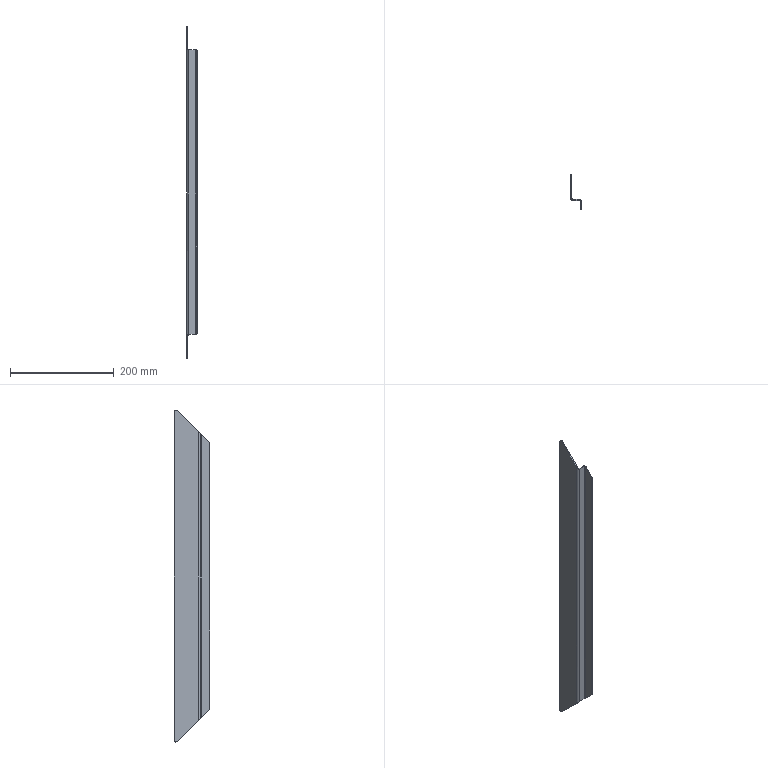Component | SolidWorks | BoxWelding-1_FrontAndRearPlate4-1 | 1 solid | 25 faces | box 20 x 68 x 641.51 mm | volume 96064 mm3 | plane 14 | cylinder 7 | spline 4 | commonest cylinder face diameters 6 x3 8 x2 4 x2
STEP:
#1=COLOUR_RGB('',0.7922,0.8196,0.9333);
#2=FILL_AREA_STYLE_COLOUR('',#1);
#3=FILL_AREA_STYLE('',(#2));
#4=SURFACE_STYLE_FILL_AREA(#3);
#5=SURFACE_SIDE_STYLE('',(#4));
#6=SURFACE_STYLE_USAGE(.BOTH.,#5);
#7=PRESENTATION_STYLE_ASSIGNMENT((#6));
#8=CARTESIAN_POINT('',(-8.991,51.201,-8.691));
#9=VERTEX_POINT('',#8);
#10=CARTESIAN_POINT('',(-8.991,51.117,-8.656));
#11=VERTEX_POINT('',#10);
#12=CARTESIAN_POINT('',(-8.991,51.201,-8.573));
#13=DIRECTION('',(-1.,-0.,-0.));
#14=DIRECTION('',(0.,0.,1.));
#15=AXIS2_PLACEMENT_3D('',#12,#13,#14);
#16=CIRCLE('',#15,0.1181);
#17=EDGE_CURVE('',#9,#11,#16,.T.);
#18=ORIENTED_EDGE('',*,*,#17,.F.);
#19=CARTESIAN_POINT('',(-8.913,51.201,-8.691));
#20=VERTEX_POINT('',#19);
#21=CARTESIAN_POINT('',(-8.991,51.201,-8.691));
#22=DIRECTION('',(1.,0.,0.));
#23=VECTOR('',#22,39.37);
#24=LINE('',#21,#23);
#25=EDGE_CURVE('',#9,#20,#24,.T.);
#26=ORIENTED_EDGE('',*,*,#25,.T.);
#27=CARTESIAN_POINT('',(-8.913,51.117,-8.656));
#28=VERTEX_POINT('',#27);
#29=CARTESIAN_POINT('',(-8.913,51.201,-8.573));
#30=DIRECTION('',(1.,0.,0.));
#31=DIRECTION('',(0.,0.,1.));
#32=AXIS2_PLACEMENT_3D('',#29,#30,#31);
#33=CIRCLE('',#32,0.1181);
#34=EDGE_CURVE('',#28,#20,#33,.T.);
#35=ORIENTED_EDGE('',*,*,#34,.F.);
#36=CARTESIAN_POINT('',(-8.913,51.117,-8.656));
#37=DIRECTION('',(1.,0.,0.));
#38=VECTOR('',#37,39.37);
#39=LINE('',#36,#38);
#40=EDGE_CURVE('',#11,#28,#39,.T.);
#41=ORIENTED_EDGE('',*,*,#40,.F.);
#42=EDGE_LOOP('',(#18,#26,#35,#41));
#43=FACE_OUTER_BOUND('',#42,.T.);
#44=CARTESIAN_POINT('',(-8.991,51.201,-8.573));
#45=DIRECTION('',(1.,0.,0.));
#46=DIRECTION('',(0.,-0.,-1.));
#47=AXIS2_PLACEMENT_3D('',#44,#45,#46);
#48=CYLINDRICAL_SURFACE('',#47,0.1181);
#49=ADVANCED_FACE('',(#43),#48,.T.);
#50=CARTESIAN_POINT('',(-8.834,49.35,14.764));
#51=VERTEX_POINT('',#50);
#52=CARTESIAN_POINT('',(-8.834,49.35,-6.889));
#53=VERTEX_POINT('',#52);
#54=CARTESIAN_POINT('',(-8.834,49.35,-8.858));
#55=DIRECTION('',(0.,-0.,-1.));
#56=VECTOR('',#55,39.37);
#57=LINE('',#54,#56);
#58=EDGE_CURVE('',#51,#53,#57,.T.);
#59=ORIENTED_EDGE('',*,*,#58,.T.);
#60=CARTESIAN_POINT('',(-8.361,49.35,-6.889));
#61=VERTEX_POINT('',#60);
#62=CARTESIAN_POINT('',(-8.913,49.35,-6.889));
#63=DIRECTION('',(-1.,-0.,-0.));
#64=VECTOR('',#63,39.37);
#65=LINE('',#62,#64);
#66=EDGE_CURVE('',#61,#53,#65,.T.);
#67=ORIENTED_EDGE('',*,*,#66,.F.);
#68=CARTESIAN_POINT('',(-8.361,49.35,14.764));
#69=VERTEX_POINT('',#68);
#70=CARTESIAN_POINT('',(-8.361,49.35,16.733));
#71=DIRECTION('',(0.,-0.,-1.));
#72=VECTOR('',#71,39.37);
#73=LINE('',#70,#72);
#74=EDGE_CURVE('',#69,#61,#73,.T.);
#75=ORIENTED_EDGE('',*,*,#74,.F.);
#76=CARTESIAN_POINT('',(-8.913,49.35,14.764));
#77=DIRECTION('',(1.,0.,0.));
#78=VECTOR('',#77,39.37);
#79=LINE('',#76,#78);
#80=EDGE_CURVE('',#51,#69,#79,.T.);
#81=ORIENTED_EDGE('',*,*,#80,.F.);
#82=EDGE_LOOP('',(#59,#67,#75,#81));
#83=FACE_OUTER_BOUND('',#82,.T.);
#84=CARTESIAN_POINT('',(-8.913,49.35,-8.858));
#85=DIRECTION('',(0.,-1.,0.));
#86=DIRECTION('',(1.,0.,0.));
#87=AXIS2_PLACEMENT_3D('',#84,#85,#86);
#88=PLANE('',#87);
#89=ADVANCED_FACE('',(#83),#88,.T.);
#90=CARTESIAN_POINT('',(-8.361,49.429,-6.889));
#91=VERTEX_POINT('',#90);
#92=CARTESIAN_POINT('',(-8.834,49.429,-6.889));
#93=VERTEX_POINT('',#92);
#94=CARTESIAN_POINT('',(-8.913,49.429,-6.889));
#95=DIRECTION('',(-1.,-0.,-0.));
#96=VECTOR('',#95,39.37);
#97=LINE('',#94,#96);
#98=EDGE_CURVE('',#91,#93,#97,.T.);
#99=ORIENTED_EDGE('',*,*,#98,.T.);
#100=CARTESIAN_POINT('',(-8.834,49.429,14.764));
#101=VERTEX_POINT('',#100);
#102=CARTESIAN_POINT('',(-8.834,49.429,16.733));
#103=DIRECTION('',(0.,-0.,-1.));
#104=VECTOR('',#103,39.37);
#105=LINE('',#102,#104);
#106=EDGE_CURVE('',#101,#93,#105,.T.);
#107=ORIENTED_EDGE('',*,*,#106,.F.);
#108=CARTESIAN_POINT('',(-8.361,49.429,14.764));
#109=VERTEX_POINT('',#108);
#110=CARTESIAN_POINT('',(-8.913,49.429,14.764));
#111=DIRECTION('',(1.,0.,0.));
#112=VECTOR('',#111,39.37);
#113=LINE('',#110,#112);
#114=EDGE_CURVE('',#101,#109,#113,.T.);
#115=ORIENTED_EDGE('',*,*,#114,.T.);
#116=CARTESIAN_POINT('',(-8.361,49.429,16.733));
#117=DIRECTION('',(0.,-0.,-1.));
#118=VECTOR('',#117,39.37);
#119=LINE('',#116,#118);
#120=EDGE_CURVE('',#109,#91,#119,.T.);
#121=ORIENTED_EDGE('',*,*,#120,.T.);
#122=EDGE_LOOP('',(#99,#107,#115,#121));
#123=FACE_OUTER_BOUND('',#122,.T.);
#124=CARTESIAN_POINT('',(-8.913,49.429,-8.858));
#125=DIRECTION('',(0.,-1.,0.));
#126=DIRECTION('',(1.,0.,0.));
#127=AXIS2_PLACEMENT_3D('',#124,#125,#126);
#128=PLANE('',#127);
#129=ADVANCED_FACE('',(#123),#128,.F.);
#130=CARTESIAN_POINT('',(-8.991,51.319,16.448));
#131=VERTEX_POINT('',#130);
#132=CARTESIAN_POINT('',(-8.991,51.319,-8.573));
#133=VERTEX_POINT('',#132);
#134=CARTESIAN_POINT('',(-8.991,51.319,-8.858));
#135=DIRECTION('',(0.,-0.,-1.));
#136=VECTOR('',#135,39.37);
#137=LINE('',#134,#136);
#138=EDGE_CURVE('',#131,#133,#137,.T.);
#139=ORIENTED_EDGE('',*,*,#138,.T.);
#140=CARTESIAN_POINT('',(-8.991,51.201,-8.573));
#141=DIRECTION('',(-1.,-0.,-0.));
#142=DIRECTION('',(0.,0.,1.));
#143=AXIS2_PLACEMENT_3D('',#140,#141,#142);
#144=CIRCLE('',#143,0.1181);
#145=EDGE_CURVE('',#133,#9,#144,.T.);
#146=ORIENTED_EDGE('',*,*,#145,.T.);
#147=ORIENTED_EDGE('',*,*,#17,.T.);
#148=CARTESIAN_POINT('',(-8.991,49.508,-7.047));
#149=VERTEX_POINT('',#148);
#150=CARTESIAN_POINT('',(-8.991,37.539,4.922));
#151=DIRECTION('',(-0.,0.7071,-0.7071));
#152=VECTOR('',#151,39.37);
#153=LINE('',#150,#152);
#154=EDGE_CURVE('',#149,#11,#153,.T.);
#155=ORIENTED_EDGE('',*,*,#154,.F.);
#156=CARTESIAN_POINT('',(-8.991,49.508,14.922));
#157=VERTEX_POINT('',#156);
#158=CARTESIAN_POINT('',(-8.991,49.508,-8.858));
#159=DIRECTION('',(-0.,0.,1.));
#160=VECTOR('',#159,39.37);
#161=LINE('',#158,#160);
#162=EDGE_CURVE('',#149,#157,#161,.T.);
#163=ORIENTED_EDGE('',*,*,#162,.T.);
#164=CARTESIAN_POINT('',(-8.991,51.117,16.531));
#165=VERTEX_POINT('',#164);
#166=CARTESIAN_POINT('',(-8.991,50.335,15.749));
#167=DIRECTION('',(0.,-0.7071,-0.7071));
#168=VECTOR('',#167,39.37);
#169=LINE('',#166,#168);
#170=EDGE_CURVE('',#165,#157,#169,.T.);
#171=ORIENTED_EDGE('',*,*,#170,.F.);
#172=CARTESIAN_POINT('',(-8.991,51.201,16.448));
#173=DIRECTION('',(-1.,-0.,-0.));
#174=DIRECTION('',(0.,0.,1.));
#175=AXIS2_PLACEMENT_3D('',#172,#173,#174);
#176=CIRCLE('',#175,0.1181);
#177=EDGE_CURVE('',#165,#131,#176,.T.);
#178=ORIENTED_EDGE('',*,*,#177,.T.);
#179=EDGE_LOOP('',(#139,#146,#147,#155,#163,#171,#178));
#180=FACE_OUTER_BOUND('',#179,.T.);
#181=CARTESIAN_POINT('',(-8.991,49.35,16.733));
#182=DIRECTION('',(-1.,-0.,-0.));
#183=DIRECTION('',(-0.,0.,1.));
#184=AXIS2_PLACEMENT_3D('',#181,#182,#183);
#185=PLANE('',#184);
#186=ADVANCED_FACE('',(#180),#185,.T.);
#187=CARTESIAN_POINT('',(-8.913,49.508,-7.047));
#188=VERTEX_POINT('',#187);
#189=CARTESIAN_POINT('',(-8.913,37.539,4.922));
#190=DIRECTION('',(-0.,0.7071,-0.7071));
#191=VECTOR('',#190,39.37);
#192=LINE('',#189,#191);
#193=EDGE_CURVE('',#188,#28,#192,.T.);
#194=ORIENTED_EDGE('',*,*,#193,.T.);
#195=ORIENTED_EDGE('',*,*,#34,.T.);
#196=CARTESIAN_POINT('',(-8.913,51.319,-8.573));
#197=VERTEX_POINT('',#196);
#198=CARTESIAN_POINT('',(-8.913,51.201,-8.573));
#199=DIRECTION('',(1.,0.,0.));
#200=DIRECTION('',(0.,0.,1.));
#201=AXIS2_PLACEMENT_3D('',#198,#199,#200);
#202=CIRCLE('',#201,0.1181);
#203=EDGE_CURVE('',#20,#197,#202,.T.);
#204=ORIENTED_EDGE('',*,*,#203,.T.);
#205=CARTESIAN_POINT('',(-8.913,51.319,16.448));
#206=VERTEX_POINT('',#205);
#207=CARTESIAN_POINT('',(-8.913,51.319,16.733));
#208=DIRECTION('',(0.,-0.,-1.));
#209=VECTOR('',#208,39.37);
#210=LINE('',#207,#209);
#211=EDGE_CURVE('',#206,#197,#210,.T.);
#212=ORIENTED_EDGE('',*,*,#211,.F.);
#213=CARTESIAN_POINT('',(-8.913,51.117,16.531));
#214=VERTEX_POINT('',#213);
#215=CARTESIAN_POINT('',(-8.913,51.201,16.448));
#216=DIRECTION('',(1.,0.,0.));
#217=DIRECTION('',(0.,0.,1.));
#218=AXIS2_PLACEMENT_3D('',#215,#216,#217);
#219=CIRCLE('',#218,0.1181);
#220=EDGE_CURVE('',#206,#214,#219,.T.);
#221=ORIENTED_EDGE('',*,*,#220,.T.);
#222=CARTESIAN_POINT('',(-8.913,49.508,14.922));
#223=VERTEX_POINT('',#222);
#224=CARTESIAN_POINT('',(-8.913,50.335,15.749));
#225=DIRECTION('',(0.,-0.7071,-0.7071));
#226=VECTOR('',#225,39.37);
#227=LINE('',#224,#226);
#228=EDGE_CURVE('',#214,#223,#227,.T.);
#229=ORIENTED_EDGE('',*,*,#228,.T.);
#230=CARTESIAN_POINT('',(-8.913,49.508,-8.858));
#231=DIRECTION('',(-0.,0.,1.));
#232=VECTOR('',#231,39.37);
#233=LINE('',#230,#232);
#234=EDGE_CURVE('',#188,#223,#233,.T.);
#235=ORIENTED_EDGE('',*,*,#234,.F.);
#236=EDGE_LOOP('',(#194,#195,#204,#212,#221,#229,#235));
#237=FACE_OUTER_BOUND('',#236,.T.);
#238=CARTESIAN_POINT('',(-8.913,49.35,16.733));
#239=DIRECTION('',(-1.,-0.,-0.));
#240=DIRECTION('',(-0.,0.,1.));
#241=AXIS2_PLACEMENT_3D('',#238,#239,#240);
#242=PLANE('',#241);
#243=ADVANCED_FACE('',(#237),#242,.F.);
#244=ORIENTED_EDGE('',*,*,#162,.F.);
#245=CARTESIAN_POINT('',(-8.834,49.35,-6.889));
#246=CARTESIAN_POINT('',(-8.926,49.35,-6.889));
#247=CARTESIAN_POINT('',(-8.991,49.416,-6.954));
#248=CARTESIAN_POINT('',(-8.991,49.508,-7.047));
#249=(BOUNDED_CURVE()B_SPLINE_CURVE(3,(#245,#246,#247,#248),.UNSPECIFIED.,.F.,.T.)B_SPLINE_CURVE_WITH_KNOTS((4,4),(3.142,4.712),.UNSPECIFIED.)CURVE()GEOMETRIC_REPRESENTATION_ITEM()RATIONAL_B_SPLINE_CURVE((1.,0.8047,0.8047,1.))REPRESENTATION_ITEM(''));
#250=EDGE_CURVE('',#53,#149,#249,.T.);
#251=ORIENTED_EDGE('',*,*,#250,.F.);
#252=ORIENTED_EDGE('',*,*,#58,.F.);
#253=CARTESIAN_POINT('',(-8.991,49.508,14.922));
#254=CARTESIAN_POINT('',(-8.991,49.416,14.83));
#255=CARTESIAN_POINT('',(-8.926,49.35,14.764));
#256=CARTESIAN_POINT('',(-8.834,49.35,14.764));
#257=(BOUNDED_CURVE()B_SPLINE_CURVE(3,(#253,#254,#255,#256),.UNSPECIFIED.,.F.,.T.)B_SPLINE_CURVE_WITH_KNOTS((4,4),(4.712,6.283),.UNSPECIFIED.)CURVE()GEOMETRIC_REPRESENTATION_ITEM()RATIONAL_B_SPLINE_CURVE((1.,0.8047,0.8047,1.))REPRESENTATION_ITEM(''));
#258=EDGE_CURVE('',#157,#51,#257,.T.);
#259=ORIENTED_EDGE('',*,*,#258,.F.);
#260=EDGE_LOOP('',(#244,#251,#252,#259));
#261=FACE_OUTER_BOUND('',#260,.T.);
#262=CARTESIAN_POINT('',(-8.834,49.508,-8.858));
#263=DIRECTION('',(0.,-0.,-1.));
#264=DIRECTION('',(0.,-1.,0.));
#265=AXIS2_PLACEMENT_3D('',#262,#263,#264);
#266=CYLINDRICAL_SURFACE('',#265,0.1575);
#267=ADVANCED_FACE('',(#261),#266,.T.);
#268=CARTESIAN_POINT('',(-8.834,49.429,-6.889));
#269=CARTESIAN_POINT('',(-8.88,49.429,-6.889));
#270=CARTESIAN_POINT('',(-8.913,49.462,-6.954));
#271=CARTESIAN_POINT('',(-8.913,49.508,-7.047));
#272=(BOUNDED_CURVE()B_SPLINE_CURVE(3,(#268,#269,#270,#271),.UNSPECIFIED.,.F.,.T.)B_SPLINE_CURVE_WITH_KNOTS((4,4),(3.142,4.712),.UNSPECIFIED.)CURVE()GEOMETRIC_REPRESENTATION_ITEM()RATIONAL_B_SPLINE_CURVE((1.,0.8047,0.8047,1.))REPRESENTATION_ITEM(''));
#273=EDGE_CURVE('',#93,#188,#272,.T.);
#274=ORIENTED_EDGE('',*,*,#273,.T.);
#275=ORIENTED_EDGE('',*,*,#234,.T.);
#276=CARTESIAN_POINT('',(-8.913,49.508,14.922));
#277=CARTESIAN_POINT('',(-8.913,49.462,14.83));
#278=CARTESIAN_POINT('',(-8.88,49.429,14.764));
#279=CARTESIAN_POINT('',(-8.834,49.429,14.764));
#280=(BOUNDED_CURVE()B_SPLINE_CURVE(3,(#276,#277,#278,#279),.UNSPECIFIED.,.F.,.T.)B_SPLINE_CURVE_WITH_KNOTS((4,4),(4.712,6.283),.UNSPECIFIED.)CURVE()GEOMETRIC_REPRESENTATION_ITEM()RATIONAL_B_SPLINE_CURVE((1.,0.8047,0.8047,1.))REPRESENTATION_ITEM(''));
#281=EDGE_CURVE('',#223,#101,#280,.T.);
#282=ORIENTED_EDGE('',*,*,#281,.T.);
#283=ORIENTED_EDGE('',*,*,#106,.T.);
#284=EDGE_LOOP('',(#274,#275,#282,#283));
#285=FACE_OUTER_BOUND('',#284,.T.);
#286=CARTESIAN_POINT('',(-8.834,49.508,-8.858));
#287=DIRECTION('',(0.,-0.,-1.));
#288=DIRECTION('',(0.,-1.,0.));
#289=AXIS2_PLACEMENT_3D('',#286,#287,#288);
#290=CYLINDRICAL_SURFACE('',#289,0.07874);
#291=ADVANCED_FACE('',(#285),#290,.F.);
#292=CARTESIAN_POINT('',(-8.204,49.272,-6.811));
#293=VERTEX_POINT('',#292);
#294=CARTESIAN_POINT('',(-8.204,49.272,14.686));
#295=VERTEX_POINT('',#294);
#296=CARTESIAN_POINT('',(-8.204,49.272,16.733));
#297=DIRECTION('',(-0.,0.,1.));
#298=VECTOR('',#297,39.37);
#299=LINE('',#296,#298);
#300=EDGE_CURVE('',#293,#295,#299,.T.);
#301=ORIENTED_EDGE('',*,*,#300,.F.);
#302=CARTESIAN_POINT('',(-8.361,49.429,-6.889));
#303=CARTESIAN_POINT('',(-8.269,49.429,-6.889));
#304=CARTESIAN_POINT('',(-8.204,49.364,-6.857));
#305=CARTESIAN_POINT('',(-8.204,49.272,-6.811));
#306=(BOUNDED_CURVE()B_SPLINE_CURVE(3,(#302,#303,#304,#305),.UNSPECIFIED.,.F.,.T.)B_SPLINE_CURVE_WITH_KNOTS((4,4),(3.142,4.712),.UNSPECIFIED.)CURVE()GEOMETRIC_REPRESENTATION_ITEM()RATIONAL_B_SPLINE_CURVE((1.,0.8047,0.8047,1.))REPRESENTATION_ITEM(''));
#307=EDGE_CURVE('',#91,#293,#306,.T.);
#308=ORIENTED_EDGE('',*,*,#307,.F.);
#309=ORIENTED_EDGE('',*,*,#120,.F.);
#310=CARTESIAN_POINT('',(-8.204,49.272,14.686));
#311=CARTESIAN_POINT('',(-8.204,49.364,14.732));
#312=CARTESIAN_POINT('',(-8.269,49.429,14.764));
#313=CARTESIAN_POINT('',(-8.361,49.429,14.764));
#314=(BOUNDED_CURVE()B_SPLINE_CURVE(3,(#310,#311,#312,#313),.UNSPECIFIED.,.F.,.T.)B_SPLINE_CURVE_WITH_KNOTS((4,4),(4.712,6.283),.UNSPECIFIED.)CURVE()GEOMETRIC_REPRESENTATION_ITEM()RATIONAL_B_SPLINE_CURVE((1.,0.8047,0.8047,1.))REPRESENTATION_ITEM(''));
#315=EDGE_CURVE('',#295,#109,#314,.T.);
#316=ORIENTED_EDGE('',*,*,#315,.F.);
#317=EDGE_LOOP('',(#301,#308,#309,#316));
#318=FACE_OUTER_BOUND('',#317,.T.);
#319=CARTESIAN_POINT('',(-8.361,49.272,16.733));
#320=DIRECTION('',(-0.,0.,1.));
#321=DIRECTION('',(1.,0.,0.));
#322=AXIS2_PLACEMENT_3D('',#319,#320,#321);
#323=CYLINDRICAL_SURFACE('',#322,0.1575);
#324=ADVANCED_FACE('',(#318),#323,.T.);
#325=CARTESIAN_POINT('',(-8.283,49.272,-6.811));
#326=VERTEX_POINT('',#325);
#327=CARTESIAN_POINT('',(-8.361,49.35,-6.889));
#328=CARTESIAN_POINT('',(-8.315,49.35,-6.889));
#329=CARTESIAN_POINT('',(-8.283,49.318,-6.857));
#330=CARTESIAN_POINT('',(-8.283,49.272,-6.811));
#331=(BOUNDED_CURVE()B_SPLINE_CURVE(3,(#327,#328,#329,#330),.UNSPECIFIED.,.F.,.T.)B_SPLINE_CURVE_WITH_KNOTS((4,4),(3.142,4.712),.UNSPECIFIED.)CURVE()GEOMETRIC_REPRESENTATION_ITEM()RATIONAL_B_SPLINE_CURVE((1.,0.8047,0.8047,1.))REPRESENTATION_ITEM(''));
#332=EDGE_CURVE('',#61,#326,#331,.T.);
#333=ORIENTED_EDGE('',*,*,#332,.T.);
#334=CARTESIAN_POINT('',(-8.283,49.272,14.686));
#335=VERTEX_POINT('',#334);
#336=CARTESIAN_POINT('',(-8.283,49.272,-8.858));
#337=DIRECTION('',(-0.,0.,1.));
#338=VECTOR('',#337,39.37);
#339=LINE('',#336,#338);
#340=EDGE_CURVE('',#326,#335,#339,.T.);
#341=ORIENTED_EDGE('',*,*,#340,.T.);
#342=CARTESIAN_POINT('',(-8.283,49.272,14.686));
#343=CARTESIAN_POINT('',(-8.283,49.318,14.732));
#344=CARTESIAN_POINT('',(-8.315,49.35,14.764));
#345=CARTESIAN_POINT('',(-8.361,49.35,14.764));
#346=(BOUNDED_CURVE()B_SPLINE_CURVE(3,(#342,#343,#344,#345),.UNSPECIFIED.,.F.,.F.)B_SPLINE_CURVE_WITH_KNOTS((4,4),(4.712,6.283),.UNSPECIFIED.)CURVE()GEOMETRIC_REPRESENTATION_ITEM()RATIONAL_B_SPLINE_CURVE((1.,0.8047,0.8047,1.))REPRESENTATION_ITEM(''));
#347=EDGE_CURVE('',#335,#69,#346,.T.);
#348=ORIENTED_EDGE('',*,*,#347,.T.);
#349=ORIENTED_EDGE('',*,*,#74,.T.);
#350=EDGE_LOOP('',(#333,#341,#348,#349));
#351=FACE_OUTER_BOUND('',#350,.T.);
#352=CARTESIAN_POINT('',(-8.361,49.272,16.733));
#353=DIRECTION('',(-0.,0.,1.));
#354=DIRECTION('',(1.,0.,0.));
#355=AXIS2_PLACEMENT_3D('',#352,#353,#354);
#356=CYLINDRICAL_SURFACE('',#355,0.07874);
#357=ADVANCED_FACE('',(#351),#356,.F.);
#358=CARTESIAN_POINT('',(-8.204,48.642,-6.181));
#359=VERTEX_POINT('',#358);
#360=CARTESIAN_POINT('',(-8.204,48.642,14.056));
#361=VERTEX_POINT('',#360);
#362=CARTESIAN_POINT('',(-8.204,48.642,16.733));
#363=DIRECTION('',(-0.,0.,1.));
#364=VECTOR('',#363,39.37);
#365=LINE('',#362,#364);
#366=EDGE_CURVE('',#359,#361,#365,.T.);
#367=ORIENTED_EDGE('',*,*,#366,.F.);
#368=CARTESIAN_POINT('',(-8.204,37.539,4.922));
#369=DIRECTION('',(0.,-0.7071,0.7071));
#370=VECTOR('',#369,39.37);
#371=LINE('',#368,#370);
#372=EDGE_CURVE('',#293,#359,#371,.T.);
#373=ORIENTED_EDGE('',*,*,#372,.F.);
#374=ORIENTED_EDGE('',*,*,#300,.T.);
#375=CARTESIAN_POINT('',(-8.204,51.319,16.733));
#376=DIRECTION('',(0.,-0.7071,-0.7071));
#377=VECTOR('',#376,39.37);
#378=LINE('',#375,#377);
#379=EDGE_CURVE('',#295,#361,#378,.T.);
#380=ORIENTED_EDGE('',*,*,#379,.T.);
#381=EDGE_LOOP('',(#367,#373,#374,#380));
#382=FACE_OUTER_BOUND('',#381,.T.);
#383=CARTESIAN_POINT('',(-8.204,49.35,16.733));
#384=DIRECTION('',(1.,0.,0.));
#385=DIRECTION('',(0.,-0.,-1.));
#386=AXIS2_PLACEMENT_3D('',#383,#384,#385);
#387=PLANE('',#386);
#388=ADVANCED_FACE('',(#382),#387,.T.);
#389=CARTESIAN_POINT('',(-8.283,48.642,-6.181));
#390=VERTEX_POINT('',#389);
#391=CARTESIAN_POINT('',(-8.283,37.539,4.922));
#392=DIRECTION('',(0.,-0.7071,0.7071));
#393=VECTOR('',#392,39.37);
#394=LINE('',#391,#393);
#395=EDGE_CURVE('',#326,#390,#394,.T.);
#396=ORIENTED_EDGE('',*,*,#395,.T.);
#397=CARTESIAN_POINT('',(-8.283,48.642,14.056));
#398=VERTEX_POINT('',#397);
#399=CARTESIAN_POINT('',(-8.283,48.642,16.733));
#400=DIRECTION('',(-0.,0.,1.));
#401=VECTOR('',#400,39.37);
#402=LINE('',#399,#401);
#403=EDGE_CURVE('',#390,#398,#402,.T.);
#404=ORIENTED_EDGE('',*,*,#403,.T.);
#405=CARTESIAN_POINT('',(-8.283,51.319,16.733));
#406=DIRECTION('',(0.,-0.7071,-0.7071));
#407=VECTOR('',#406,39.37);
#408=LINE('',#405,#407);
#409=EDGE_CURVE('',#335,#398,#408,.T.);
#410=ORIENTED_EDGE('',*,*,#409,.F.);
#411=ORIENTED_EDGE('',*,*,#340,.F.);
#412=EDGE_LOOP('',(#396,#404,#410,#411));
#413=FACE_OUTER_BOUND('',#412,.T.);
#414=CARTESIAN_POINT('',(-8.283,49.35,16.733));
#415=DIRECTION('',(1.,0.,0.));
#416=DIRECTION('',(0.,-0.,-1.));
#417=AXIS2_PLACEMENT_3D('',#414,#415,#416);
#418=PLANE('',#417);
#419=ADVANCED_FACE('',(#413),#418,.F.);
#420=ORIENTED_EDGE('',*,*,#403,.F.);
#421=CARTESIAN_POINT('',(-8.283,48.642,-6.181));
#422=DIRECTION('',(1.,0.,0.));
#423=VECTOR('',#422,39.37);
#424=LINE('',#421,#423);
#425=EDGE_CURVE('',#390,#359,#424,.T.);
#426=ORIENTED_EDGE('',*,*,#425,.T.);
#427=ORIENTED_EDGE('',*,*,#366,.T.);
#428=CARTESIAN_POINT('',(-8.204,48.642,14.056));
#429=DIRECTION('',(-1.,-0.,-0.));
#430=VECTOR('',#429,39.37);
#431=LINE('',#428,#430);
#432=EDGE_CURVE('',#361,#398,#431,.T.);
#433=ORIENTED_EDGE('',*,*,#432,.T.);
#434=EDGE_LOOP('',(#420,#426,#427,#433));
#435=FACE_OUTER_BOUND('',#434,.T.);
#436=CARTESIAN_POINT('',(-8.204,48.642,16.733));
#437=DIRECTION('',(0.,-1.,0.));
#438=DIRECTION('',(1.,0.,0.));
#439=AXIS2_PLACEMENT_3D('',#436,#437,#438);
#440=PLANE('',#439);
#441=ADVANCED_FACE('',(#435),#440,.T.);
#442=ORIENTED_EDGE('',*,*,#211,.T.);
#443=CARTESIAN_POINT('',(-8.991,51.319,-8.573));
#444=DIRECTION('',(-1.,-0.,-0.));
#445=VECTOR('',#444,39.37);
#446=LINE('',#443,#445);
#447=EDGE_CURVE('',#197,#133,#446,.T.);
#448=ORIENTED_EDGE('',*,*,#447,.T.);
#449=ORIENTED_EDGE('',*,*,#138,.F.);
#450=CARTESIAN_POINT('',(-8.991,51.319,16.448));
#451=DIRECTION('',(1.,0.,0.));
#452=VECTOR('',#451,39.37);
#453=LINE('',#450,#452);
#454=EDGE_CURVE('',#131,#206,#453,.T.);
#455=ORIENTED_EDGE('',*,*,#454,.T.);
#456=EDGE_LOOP('',(#442,#448,#449,#455));
#457=FACE_OUTER_BOUND('',#456,.T.);
#458=CARTESIAN_POINT('',(-8.991,51.319,-8.858));
#459=DIRECTION('',(-0.,1.,-0.));
#460=DIRECTION('',(0.,-0.,-1.));
#461=AXIS2_PLACEMENT_3D('',#458,#459,#460);
#462=PLANE('',#461);
#463=ADVANCED_FACE('',(#457),#462,.T.);
#464=ORIENTED_EDGE('',*,*,#228,.F.);
#465=CARTESIAN_POINT('',(-8.913,51.117,16.531));
#466=DIRECTION('',(-1.,-0.,-0.));
#467=VECTOR('',#466,39.37);
#468=LINE('',#465,#467);
#469=EDGE_CURVE('',#214,#165,#468,.T.);
#470=ORIENTED_EDGE('',*,*,#469,.T.);
#471=ORIENTED_EDGE('',*,*,#170,.T.);
#472=CARTESIAN_POINT('',(-8.913,49.508,14.922));
#473=DIRECTION('',(-1.,-0.,-0.));
#474=VECTOR('',#473,39.37);
#475=LINE('',#472,#474);
#476=EDGE_CURVE('',#223,#157,#475,.T.);
#477=ORIENTED_EDGE('',*,*,#476,.F.);
#478=EDGE_LOOP('',(#464,#470,#471,#477));
#479=FACE_OUTER_BOUND('',#478,.T.);
#480=CARTESIAN_POINT('',(-8.913,50.335,15.749));
#481=DIRECTION('',(-0.,0.7071,-0.7071));
#482=DIRECTION('',(0.,-0.7071,-0.7071));
#483=AXIS2_PLACEMENT_3D('',#480,#481,#482);
#484=PLANE('',#483);
#485=ADVANCED_FACE('',(#479),#484,.F.);
#486=ORIENTED_EDGE('',*,*,#80,.T.);
#487=CARTESIAN_POINT('',(-8.361,49.35,14.764));
#488=DIRECTION('',(-0.,1.,-0.));
#489=VECTOR('',#488,39.37);
#490=LINE('',#487,#489);
#491=EDGE_CURVE('',#69,#109,#490,.T.);
#492=ORIENTED_EDGE('',*,*,#491,.T.);
#493=ORIENTED_EDGE('',*,*,#114,.F.);
#494=CARTESIAN_POINT('',(-8.834,49.35,14.764));
#495=DIRECTION('',(-0.,1.,-0.));
#496=VECTOR('',#495,39.37);
#497=LINE('',#494,#496);
#498=EDGE_CURVE('',#51,#101,#497,.T.);
#499=ORIENTED_EDGE('',*,*,#498,.F.);
#500=EDGE_LOOP('',(#486,#492,#493,#499));
#501=FACE_OUTER_BOUND('',#500,.T.);
#502=CARTESIAN_POINT('',(-8.913,49.35,14.764));
#503=DIRECTION('',(0.,-0.,-1.));
#504=DIRECTION('',(1.,0.,0.));
#505=AXIS2_PLACEMENT_3D('',#502,#503,#504);
#506=PLANE('',#505);
#507=ADVANCED_FACE('',(#501),#506,.F.);
#508=ORIENTED_EDGE('',*,*,#379,.F.);
#509=CARTESIAN_POINT('',(-8.204,49.272,14.686));
#510=DIRECTION('',(-1.,-0.,-0.));
#511=VECTOR('',#510,39.37);
#512=LINE('',#509,#511);
#513=EDGE_CURVE('',#295,#335,#512,.T.);
#514=ORIENTED_EDGE('',*,*,#513,.T.);
#515=ORIENTED_EDGE('',*,*,#409,.T.);
#516=ORIENTED_EDGE('',*,*,#432,.F.);
#517=EDGE_LOOP('',(#508,#514,#515,#516));
#518=FACE_OUTER_BOUND('',#517,.T.);
#519=CARTESIAN_POINT('',(-8.204,51.319,16.733));
#520=DIRECTION('',(0.,-0.7071,0.7071));
#521=DIRECTION('',(0.,-0.7071,-0.7071));
#522=AXIS2_PLACEMENT_3D('',#519,#520,#521);
#523=PLANE('',#522);
#524=ADVANCED_FACE('',(#518),#523,.T.);
#525=ORIENTED_EDGE('',*,*,#491,.F.);
#526=ORIENTED_EDGE('',*,*,#347,.F.);
#527=ORIENTED_EDGE('',*,*,#513,.F.);
#528=ORIENTED_EDGE('',*,*,#315,.T.);
#529=EDGE_LOOP('',(#525,#526,#527,#528));
#530=FACE_OUTER_BOUND('',#529,.T.);
#531=CARTESIAN_POINT('',(-8.361,49.429,14.764));
#532=CARTESIAN_POINT('',(-8.361,49.403,14.764));
#533=CARTESIAN_POINT('',(-8.361,49.377,14.764));
#534=CARTESIAN_POINT('',(-8.361,49.35,14.764));
#535=CARTESIAN_POINT('',(-8.676,49.429,14.764));
#536=CARTESIAN_POINT('',(-8.624,49.403,14.764));
#537=CARTESIAN_POINT('',(-8.571,49.377,14.764));
#538=CARTESIAN_POINT('',(-8.519,49.35,14.764));
#539=CARTESIAN_POINT('',(-8.676,49.114,14.607));
#540=CARTESIAN_POINT('',(-8.624,49.14,14.607));
#541=CARTESIAN_POINT('',(-8.571,49.167,14.607));
#542=CARTESIAN_POINT('',(-8.519,49.193,14.607));
#543=CARTESIAN_POINT('',(-8.361,49.114,14.607));
#544=CARTESIAN_POINT('',(-8.361,49.14,14.607));
#545=CARTESIAN_POINT('',(-8.361,49.167,14.607));
#546=CARTESIAN_POINT('',(-8.361,49.193,14.607));
#547=CARTESIAN_POINT('',(-8.046,49.114,14.607));
#548=CARTESIAN_POINT('',(-8.099,49.14,14.607));
#549=CARTESIAN_POINT('',(-8.151,49.167,14.607));
#550=CARTESIAN_POINT('',(-8.204,49.193,14.607));
#551=CARTESIAN_POINT('',(-8.046,49.429,14.764));
#552=CARTESIAN_POINT('',(-8.099,49.403,14.764));
#553=CARTESIAN_POINT('',(-8.151,49.377,14.764));
#554=CARTESIAN_POINT('',(-8.204,49.35,14.764));
#555=CARTESIAN_POINT('',(-8.361,49.429,14.764));
#556=CARTESIAN_POINT('',(-8.361,49.403,14.764));
#557=CARTESIAN_POINT('',(-8.361,49.377,14.764));
#558=CARTESIAN_POINT('',(-8.361,49.35,14.764));
#559=(BOUNDED_SURFACE()B_SPLINE_SURFACE(3,3,((#531,#532,#533,#534),(#535,#536,#537,#538),(#539,#540,#541,#542),(#543,#544,#545,#546),(#547,#548,#549,#550),(#551,#552,#553,#554),(#555,#556,#557,#558)),.UNSPECIFIED.,.T.,.F.,.F.)B_SPLINE_SURFACE_WITH_KNOTS((4,3,4),(4,4),(0.,0.5,1.),(0.,1.),.UNSPECIFIED.)GEOMETRIC_REPRESENTATION_ITEM()RATIONAL_B_SPLINE_SURFACE(((1.,1.,1.,1.),(0.3333,0.3333,0.3333,0.3333),(0.3333,0.3333,0.3333,0.3333),(1.,1.,1.,1.),(0.3333,0.3333,0.3333,0.3333),(0.3333,0.3333,0.3333,0.3333),(1.,1.,1.,1.)))REPRESENTATION_ITEM('')SURFACE());
#560=ADVANCED_FACE('',(#530),#559,.T.);
#561=ORIENTED_EDGE('',*,*,#258,.T.);
#562=ORIENTED_EDGE('',*,*,#498,.T.);
#563=ORIENTED_EDGE('',*,*,#281,.F.);
#564=ORIENTED_EDGE('',*,*,#476,.T.);
#565=EDGE_LOOP('',(#561,#562,#563,#564));
#566=FACE_OUTER_BOUND('',#565,.T.);
#567=CARTESIAN_POINT('',(-8.834,49.35,14.764));
#568=CARTESIAN_POINT('',(-8.834,49.377,14.764));
#569=CARTESIAN_POINT('',(-8.834,49.403,14.764));
#570=CARTESIAN_POINT('',(-8.834,49.429,14.764));
#571=CARTESIAN_POINT('',(-8.519,49.35,14.764));
#572=CARTESIAN_POINT('',(-8.571,49.377,14.764));
#573=CARTESIAN_POINT('',(-8.624,49.403,14.764));
#574=CARTESIAN_POINT('',(-8.676,49.429,14.764));
#575=CARTESIAN_POINT('',(-8.519,49.665,15.079));
#576=CARTESIAN_POINT('',(-8.571,49.639,15.079));
#577=CARTESIAN_POINT('',(-8.624,49.613,15.079));
#578=CARTESIAN_POINT('',(-8.676,49.587,15.079));
#579=CARTESIAN_POINT('',(-8.834,49.665,15.079));
#580=CARTESIAN_POINT('',(-8.834,49.639,15.079));
#581=CARTESIAN_POINT('',(-8.834,49.613,15.079));
#582=CARTESIAN_POINT('',(-8.834,49.587,15.079));
#583=CARTESIAN_POINT('',(-9.149,49.665,15.079));
#584=CARTESIAN_POINT('',(-9.096,49.639,15.079));
#585=CARTESIAN_POINT('',(-9.044,49.613,15.079));
#586=CARTESIAN_POINT('',(-8.991,49.587,15.079));
#587=CARTESIAN_POINT('',(-9.149,49.35,14.764));
#588=CARTESIAN_POINT('',(-9.096,49.377,14.764));
#589=CARTESIAN_POINT('',(-9.044,49.403,14.764));
#590=CARTESIAN_POINT('',(-8.991,49.429,14.764));
#591=CARTESIAN_POINT('',(-8.834,49.35,14.764));
#592=CARTESIAN_POINT('',(-8.834,49.377,14.764));
#593=CARTESIAN_POINT('',(-8.834,49.403,14.764));
#594=CARTESIAN_POINT('',(-8.834,49.429,14.764));
#595=(BOUNDED_SURFACE()B_SPLINE_SURFACE(3,3,((#567,#568,#569,#570),(#571,#572,#573,#574),(#575,#576,#577,#578),(#579,#580,#581,#582),(#583,#584,#585,#586),(#587,#588,#589,#590),(#591,#592,#593,#594)),.UNSPECIFIED.,.T.,.F.,.F.)B_SPLINE_SURFACE_WITH_KNOTS((4,3,4),(4,4),(0.,0.5,1.),(0.,1.),.UNSPECIFIED.)GEOMETRIC_REPRESENTATION_ITEM()RATIONAL_B_SPLINE_SURFACE(((1.,1.,1.,1.),(0.3333,0.3333,0.3333,0.3333),(0.3333,0.3333,0.3333,0.3333),(1.,1.,1.,1.),(0.3333,0.3333,0.3333,0.3333),(0.3333,0.3333,0.3333,0.3333),(1.,1.,1.,1.)))REPRESENTATION_ITEM('')SURFACE());
#596=ADVANCED_FACE('',(#566),#595,.T.);
#597=ORIENTED_EDGE('',*,*,#154,.T.);
#598=ORIENTED_EDGE('',*,*,#40,.T.);
#599=ORIENTED_EDGE('',*,*,#193,.F.);
#600=CARTESIAN_POINT('',(-8.913,49.508,-7.047));
#601=DIRECTION('',(-1.,-0.,-0.));
#602=VECTOR('',#601,39.37);
#603=LINE('',#600,#602);
#604=EDGE_CURVE('',#188,#149,#603,.T.);
#605=ORIENTED_EDGE('',*,*,#604,.T.);
#606=EDGE_LOOP('',(#597,#598,#599,#605));
#607=FACE_OUTER_BOUND('',#606,.T.);
#608=CARTESIAN_POINT('',(-8.913,37.539,4.922));
#609=DIRECTION('',(-0.,0.7071,0.7071));
#610=DIRECTION('',(-0.,0.7071,-0.7071));
#611=AXIS2_PLACEMENT_3D('',#608,#609,#610);
#612=PLANE('',#611);
#613=ADVANCED_FACE('',(#607),#612,.F.);
#614=ORIENTED_EDGE('',*,*,#66,.T.);
#615=CARTESIAN_POINT('',(-8.834,49.35,-6.889));
#616=DIRECTION('',(-0.,1.,-0.));
#617=VECTOR('',#616,39.37);
#618=LINE('',#615,#617);
#619=EDGE_CURVE('',#53,#93,#618,.T.);
#620=ORIENTED_EDGE('',*,*,#619,.T.);
#621=ORIENTED_EDGE('',*,*,#98,.F.);
#622=CARTESIAN_POINT('',(-8.361,49.35,-6.889));
#623=DIRECTION('',(-0.,1.,-0.));
#624=VECTOR('',#623,39.37);
#625=LINE('',#622,#624);
#626=EDGE_CURVE('',#61,#91,#625,.T.);
#627=ORIENTED_EDGE('',*,*,#626,.F.);
#628=EDGE_LOOP('',(#614,#620,#621,#627));
#629=FACE_OUTER_BOUND('',#628,.T.);
#630=CARTESIAN_POINT('',(-8.913,49.35,-6.889));
#631=DIRECTION('',(-0.,0.,1.));
#632=DIRECTION('',(-1.,-0.,-0.));
#633=AXIS2_PLACEMENT_3D('',#630,#631,#632);
#634=PLANE('',#633);
#635=ADVANCED_FACE('',(#629),#634,.F.);
#636=ORIENTED_EDGE('',*,*,#425,.F.);
#637=ORIENTED_EDGE('',*,*,#395,.F.);
#638=CARTESIAN_POINT('',(-8.283,49.272,-6.811));
#639=DIRECTION('',(1.,0.,0.));
#640=VECTOR('',#639,39.37);
#641=LINE('',#638,#640);
#642=EDGE_CURVE('',#326,#293,#641,.T.);
#643=ORIENTED_EDGE('',*,*,#642,.T.);
#644=ORIENTED_EDGE('',*,*,#372,.T.);
#645=EDGE_LOOP('',(#636,#637,#643,#644));
#646=FACE_OUTER_BOUND('',#645,.T.);
#647=CARTESIAN_POINT('',(-8.283,37.539,4.922));
#648=DIRECTION('',(-0.,0.7071,0.7071));
#649=DIRECTION('',(0.,-0.7071,0.7071));
#650=AXIS2_PLACEMENT_3D('',#647,#648,#649);
#651=PLANE('',#650);
#652=ADVANCED_FACE('',(#646),#651,.F.);
#653=ORIENTED_EDGE('',*,*,#642,.F.);
#654=ORIENTED_EDGE('',*,*,#332,.F.);
#655=ORIENTED_EDGE('',*,*,#626,.T.);
#656=ORIENTED_EDGE('',*,*,#307,.T.);
#657=EDGE_LOOP('',(#653,#654,#655,#656));
#658=FACE_OUTER_BOUND('',#657,.T.);
#659=CARTESIAN_POINT('',(-8.361,49.114,-6.732));
#660=CARTESIAN_POINT('',(-8.361,49.14,-6.732));
#661=CARTESIAN_POINT('',(-8.361,49.167,-6.732));
#662=CARTESIAN_POINT('',(-8.361,49.193,-6.732));
#663=CARTESIAN_POINT('',(-8.676,49.114,-6.732));
#664=CARTESIAN_POINT('',(-8.624,49.14,-6.732));
#665=CARTESIAN_POINT('',(-8.571,49.167,-6.732));
#666=CARTESIAN_POINT('',(-8.519,49.193,-6.732));
#667=CARTESIAN_POINT('',(-8.676,49.429,-6.889));
#668=CARTESIAN_POINT('',(-8.624,49.403,-6.889));
#669=CARTESIAN_POINT('',(-8.571,49.377,-6.889));
#670=CARTESIAN_POINT('',(-8.519,49.35,-6.889));
#671=CARTESIAN_POINT('',(-8.361,49.429,-6.889));
#672=CARTESIAN_POINT('',(-8.361,49.403,-6.889));
#673=CARTESIAN_POINT('',(-8.361,49.377,-6.889));
#674=CARTESIAN_POINT('',(-8.361,49.35,-6.889));
#675=CARTESIAN_POINT('',(-8.046,49.429,-6.889));
#676=CARTESIAN_POINT('',(-8.099,49.403,-6.889));
#677=CARTESIAN_POINT('',(-8.151,49.377,-6.889));
#678=CARTESIAN_POINT('',(-8.204,49.35,-6.889));
#679=CARTESIAN_POINT('',(-8.046,49.114,-6.732));
#680=CARTESIAN_POINT('',(-8.099,49.14,-6.732));
#681=CARTESIAN_POINT('',(-8.151,49.167,-6.732));
#682=CARTESIAN_POINT('',(-8.204,49.193,-6.732));
#683=CARTESIAN_POINT('',(-8.361,49.114,-6.732));
#684=CARTESIAN_POINT('',(-8.361,49.14,-6.732));
#685=CARTESIAN_POINT('',(-8.361,49.167,-6.732));
#686=CARTESIAN_POINT('',(-8.361,49.193,-6.732));
#687=(BOUNDED_SURFACE()B_SPLINE_SURFACE(3,3,((#659,#660,#661,#662),(#663,#664,#665,#666),(#667,#668,#669,#670),(#671,#672,#673,#674),(#675,#676,#677,#678),(#679,#680,#681,#682),(#683,#684,#685,#686)),.UNSPECIFIED.,.T.,.F.,.F.)B_SPLINE_SURFACE_WITH_KNOTS((4,3,4),(4,4),(0.,0.5,1.),(0.,1.),.UNSPECIFIED.)GEOMETRIC_REPRESENTATION_ITEM()RATIONAL_B_SPLINE_SURFACE(((1.,1.,1.,1.),(0.3333,0.3333,0.3333,0.3333),(0.3333,0.3333,0.3333,0.3333),(1.,1.,1.,1.),(0.3333,0.3333,0.3333,0.3333),(0.3333,0.3333,0.3333,0.3333),(1.,1.,1.,1.)))REPRESENTATION_ITEM('')SURFACE());
#688=ADVANCED_FACE('',(#658),#687,.T.);
#689=ORIENTED_EDGE('',*,*,#250,.T.);
#690=ORIENTED_EDGE('',*,*,#604,.F.);
#691=ORIENTED_EDGE('',*,*,#273,.F.);
#692=ORIENTED_EDGE('',*,*,#619,.F.);
#693=EDGE_LOOP('',(#689,#690,#691,#692));
#694=FACE_OUTER_BOUND('',#693,.T.);
#695=CARTESIAN_POINT('',(-8.834,49.665,-7.204));
#696=CARTESIAN_POINT('',(-8.834,49.639,-7.204));
#697=CARTESIAN_POINT('',(-8.834,49.613,-7.204));
#698=CARTESIAN_POINT('',(-8.834,49.587,-7.204));
#699=CARTESIAN_POINT('',(-8.519,49.665,-7.204));
#700=CARTESIAN_POINT('',(-8.571,49.639,-7.204));
#701=CARTESIAN_POINT('',(-8.624,49.613,-7.204));
#702=CARTESIAN_POINT('',(-8.676,49.587,-7.204));
#703=CARTESIAN_POINT('',(-8.519,49.35,-6.889));
#704=CARTESIAN_POINT('',(-8.571,49.377,-6.889));
#705=CARTESIAN_POINT('',(-8.624,49.403,-6.889));
#706=CARTESIAN_POINT('',(-8.676,49.429,-6.889));
#707=CARTESIAN_POINT('',(-8.834,49.35,-6.889));
#708=CARTESIAN_POINT('',(-8.834,49.377,-6.889));
#709=CARTESIAN_POINT('',(-8.834,49.403,-6.889));
#710=CARTESIAN_POINT('',(-8.834,49.429,-6.889));
#711=CARTESIAN_POINT('',(-9.149,49.35,-6.889));
#712=CARTESIAN_POINT('',(-9.096,49.377,-6.889));
#713=CARTESIAN_POINT('',(-9.044,49.403,-6.889));
#714=CARTESIAN_POINT('',(-8.991,49.429,-6.889));
#715=CARTESIAN_POINT('',(-9.149,49.665,-7.204));
#716=CARTESIAN_POINT('',(-9.096,49.639,-7.204));
#717=CARTESIAN_POINT('',(-9.044,49.613,-7.204));
#718=CARTESIAN_POINT('',(-8.991,49.587,-7.204));
#719=CARTESIAN_POINT('',(-8.834,49.665,-7.204));
#720=CARTESIAN_POINT('',(-8.834,49.639,-7.204));
#721=CARTESIAN_POINT('',(-8.834,49.613,-7.204));
#722=CARTESIAN_POINT('',(-8.834,49.587,-7.204));
#723=(BOUNDED_SURFACE()B_SPLINE_SURFACE(3,3,((#695,#696,#697,#698),(#699,#700,#701,#702),(#703,#704,#705,#706),(#707,#708,#709,#710),(#711,#712,#713,#714),(#715,#716,#717,#718),(#719,#720,#721,#722)),.UNSPECIFIED.,.T.,.F.,.F.)B_SPLINE_SURFACE_WITH_KNOTS((4,3,4),(4,4),(0.,0.5,1.),(0.,1.),.UNSPECIFIED.)GEOMETRIC_REPRESENTATION_ITEM()RATIONAL_B_SPLINE_SURFACE(((1.,1.,1.,1.),(0.3333,0.3333,0.3333,0.3333),(0.3333,0.3333,0.3333,0.3333),(1.,1.,1.,1.),(0.3333,0.3333,0.3333,0.3333),(0.3333,0.3333,0.3333,0.3333),(1.,1.,1.,1.)))REPRESENTATION_ITEM('')SURFACE());
#724=ADVANCED_FACE('',(#694),#723,.T.);
#725=ORIENTED_EDGE('',*,*,#25,.F.);
#726=ORIENTED_EDGE('',*,*,#145,.F.);
#727=ORIENTED_EDGE('',*,*,#447,.F.);
#728=ORIENTED_EDGE('',*,*,#203,.F.);
#729=EDGE_LOOP('',(#725,#726,#727,#728));
#730=FACE_OUTER_BOUND('',#729,.T.);
#731=CARTESIAN_POINT('',(-8.991,51.201,-8.573));
#732=DIRECTION('',(1.,0.,0.));
#733=DIRECTION('',(0.,-0.,-1.));
#734=AXIS2_PLACEMENT_3D('',#731,#732,#733);
#735=CYLINDRICAL_SURFACE('',#734,0.1181);
#736=ADVANCED_FACE('',(#730),#735,.T.);
#737=ORIENTED_EDGE('',*,*,#220,.F.);
#738=ORIENTED_EDGE('',*,*,#454,.F.);
#739=ORIENTED_EDGE('',*,*,#177,.F.);
#740=ORIENTED_EDGE('',*,*,#469,.F.);
#741=EDGE_LOOP('',(#737,#738,#739,#740));
#742=FACE_OUTER_BOUND('',#741,.T.);
#743=CARTESIAN_POINT('',(-8.913,51.201,16.448));
#744=DIRECTION('',(1.,0.,0.));
#745=DIRECTION('',(0.,-0.,-1.));
#746=AXIS2_PLACEMENT_3D('',#743,#744,#745);
#747=CYLINDRICAL_SURFACE('',#746,0.1181);
#748=ADVANCED_FACE('',(#742),#747,.T.);
#749=CLOSED_SHELL('',(#49,#89,#129,#186,#243,#267,#291,#324,#357,#388,#419,#441,#463,#485,#507,#524,#560,#596,#613,#635,#652,#688,#724,#736,#748));
#750=MANIFOLD_SOLID_BREP('',#749);
#751=STYLED_ITEM('',(#7),#750);
#752=(LENGTH_UNIT()NAMED_UNIT(*)SI_UNIT($,.METRE.));
#753=LENGTH_MEASURE_WITH_UNIT(LENGTH_MEASURE(0.0254),#752);
#754=DIMENSIONAL_EXPONENTS(1.,0.,0.,0.,0.,0.,0.);
#755=(CONVERSION_BASED_UNIT('',#753)LENGTH_UNIT()NAMED_UNIT(#754));
#756=UNCERTAINTY_MEASURE_WITH_UNIT(LENGTH_MEASURE(0.00001),#755,'','');
#757=(NAMED_UNIT(*)PLANE_ANGLE_UNIT()SI_UNIT($,.RADIAN.));
#758=(NAMED_UNIT(*)SI_UNIT($,.STERADIAN.)SOLID_ANGLE_UNIT());
#759=(GEOMETRIC_REPRESENTATION_CONTEXT(3)GLOBAL_UNCERTAINTY_ASSIGNED_CONTEXT((#756))GLOBAL_UNIT_ASSIGNED_CONTEXT((#755,#757,#758))REPRESENTATION_CONTEXT('',''));
#760=MECHANICAL_DESIGN_GEOMETRIC_PRESENTATION_REPRESENTATION('',(#751),#759);
#761=PRESENTATION_LAYER_ASSIGNMENT('','',(#751));
#762=CARTESIAN_POINT('',(0.,0.,0.));
#763=DIRECTION('',(0.,0.,1.));
#764=DIRECTION('',(1.,0.,0.));
#765=AXIS2_PLACEMENT_3D('',#762,#763,#764);
#766=(LENGTH_UNIT()NAMED_UNIT(*)SI_UNIT($,.METRE.));
#767=LENGTH_MEASURE_WITH_UNIT(LENGTH_MEASURE(0.0254),#766);
#768=DIMENSIONAL_EXPONENTS(1.,0.,0.,0.,0.,0.,0.);
#769=(CONVERSION_BASED_UNIT('',#767)LENGTH_UNIT()NAMED_UNIT(#768));
#770=UNCERTAINTY_MEASURE_WITH_UNIT(LENGTH_MEASURE(0.00001),#769,'','');
#771=(NAMED_UNIT(*)PLANE_ANGLE_UNIT()SI_UNIT($,.RADIAN.));
#772=(NAMED_UNIT(*)SI_UNIT($,.STERADIAN.)SOLID_ANGLE_UNIT());
#773=(GEOMETRIC_REPRESENTATION_CONTEXT(3)GLOBAL_UNCERTAINTY_ASSIGNED_CONTEXT((#770))GLOBAL_UNIT_ASSIGNED_CONTEXT((#769,#771,#772))REPRESENTATION_CONTEXT('',''));
#774=ADVANCED_BREP_SHAPE_REPRESENTATION('',(#750,#765),#773);